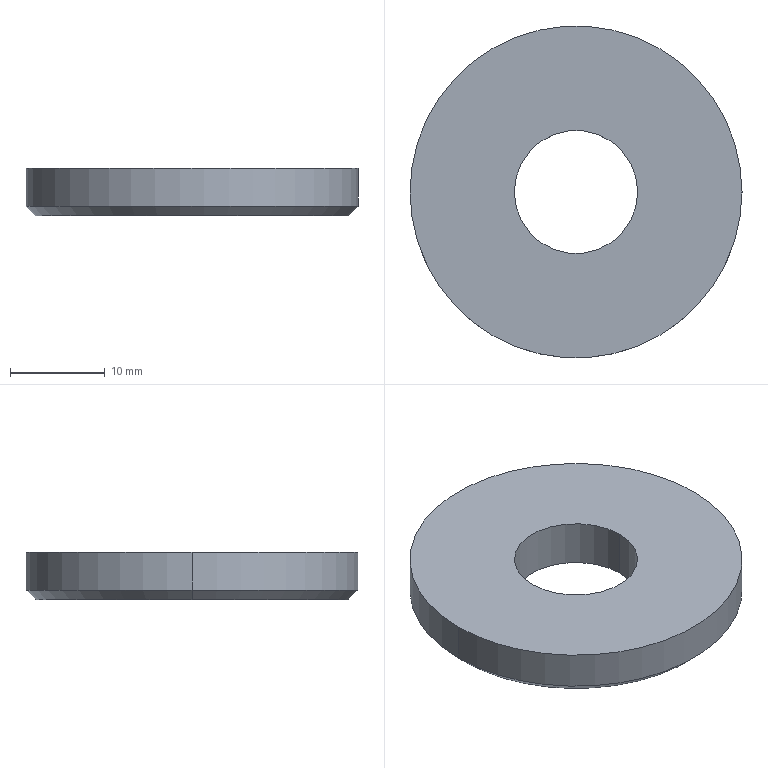Component | SolidWorks | DoubleFilmTransport-1_TensionConnectionAxisPad-1 | 1 solid | 8 faces | box 35 x 35 x 5 mm | volume 4093 mm3 | cylinder 4 | cone 2 | plane 2 | commonest cylinder face diameters 13 x2 35 x2
build123d program:
from build123d import *


with BuildPart() as part:
    # Sketch1 → Revolve1 (revolve)
    with BuildSketch(Plane.XY, mode=Mode.PRIVATE) as revolve1_sk:
        Polygon((5, 16.5), (4, 17.5), (0, 17.5), (0, 6.5), (5, 6.5), align=None)
    revolve(revolve1_sk.sketch.rotate(Axis((0, 0, 0), (1, 0, 0)), 270), axis=Axis((0, 0, 0), (1, 0, 0)))


solid = part.part

# Placed as in the assembly
solid = solid.moved(Location((-384.677, 265.373, 76), (0, 90, 0)))
STEP:
#1=COLOUR_RGB('',0.7922,0.8196,0.9333);
#2=FILL_AREA_STYLE_COLOUR('',#1);
#3=FILL_AREA_STYLE('',(#2));
#4=SURFACE_STYLE_FILL_AREA(#3);
#5=SURFACE_SIDE_STYLE('',(#4));
#6=SURFACE_STYLE_USAGE(.BOTH.,#5);
#7=PRESENTATION_STYLE_ASSIGNMENT((#6));
#8=CARTESIAN_POINT('',(-14.889,10.448,2.992));
#9=VERTEX_POINT('',#8);
#10=CARTESIAN_POINT('',(-15.401,10.448,2.992));
#11=VERTEX_POINT('',#10);
#12=CARTESIAN_POINT('',(-15.145,10.448,2.992));
#13=DIRECTION('',(0.,0.,-1.));
#14=DIRECTION('',(-1.,0.,0.));
#15=AXIS2_PLACEMENT_3D('',#12,#13,#14);
#16=CIRCLE('',#15,0.2559);
#17=EDGE_CURVE('',#9,#11,#16,.T.);
#18=ORIENTED_EDGE('',*,*,#17,.F.);
#19=CARTESIAN_POINT('',(-14.889,10.448,2.795));
#20=VERTEX_POINT('',#19);
#21=CARTESIAN_POINT('',(-14.889,10.448,2.992));
#22=DIRECTION('',(0.,0.,-1.));
#23=VECTOR('',#22,39.37);
#24=LINE('',#21,#23);
#25=EDGE_CURVE('',#9,#20,#24,.T.);
#26=ORIENTED_EDGE('',*,*,#25,.T.);
#27=CARTESIAN_POINT('',(-15.401,10.448,2.795));
#28=VERTEX_POINT('',#27);
#29=CARTESIAN_POINT('',(-15.145,10.448,2.795));
#30=DIRECTION('',(0.,0.,-1.));
#31=DIRECTION('',(-1.,0.,0.));
#32=AXIS2_PLACEMENT_3D('',#29,#30,#31);
#33=CIRCLE('',#32,0.2559);
#34=EDGE_CURVE('',#20,#28,#33,.T.);
#35=ORIENTED_EDGE('',*,*,#34,.T.);
#36=CARTESIAN_POINT('',(-15.401,10.448,2.992));
#37=DIRECTION('',(0.,0.,-1.));
#38=VECTOR('',#37,39.37);
#39=LINE('',#36,#38);
#40=EDGE_CURVE('',#11,#28,#39,.T.);
#41=ORIENTED_EDGE('',*,*,#40,.F.);
#42=EDGE_LOOP('',(#18,#26,#35,#41));
#43=FACE_OUTER_BOUND('',#42,.T.);
#44=CARTESIAN_POINT('',(-15.145,10.448,2.992));
#45=DIRECTION('',(0.,0.,-1.));
#46=DIRECTION('',(-1.,0.,0.));
#47=AXIS2_PLACEMENT_3D('',#44,#45,#46);
#48=CYLINDRICAL_SURFACE('',#47,0.2559);
#49=ADVANCED_FACE('',(#43),#48,.F.);
#50=CARTESIAN_POINT('',(-15.834,10.448,2.992));
#51=VERTEX_POINT('',#50);
#52=CARTESIAN_POINT('',(-14.456,10.448,2.992));
#53=VERTEX_POINT('',#52);
#54=CARTESIAN_POINT('',(-15.145,10.448,2.992));
#55=DIRECTION('',(0.,0.,-1.));
#56=DIRECTION('',(-1.,0.,0.));
#57=AXIS2_PLACEMENT_3D('',#54,#55,#56);
#58=CIRCLE('',#57,0.689);
#59=EDGE_CURVE('',#51,#53,#58,.T.);
#60=ORIENTED_EDGE('',*,*,#59,.T.);
#61=CARTESIAN_POINT('',(-14.456,10.448,2.835));
#62=VERTEX_POINT('',#61);
#63=CARTESIAN_POINT('',(-14.456,10.448,2.992));
#64=DIRECTION('',(0.,0.,-1.));
#65=VECTOR('',#64,39.37);
#66=LINE('',#63,#65);
#67=EDGE_CURVE('',#53,#62,#66,.T.);
#68=ORIENTED_EDGE('',*,*,#67,.T.);
#69=CARTESIAN_POINT('',(-15.834,10.448,2.835));
#70=VERTEX_POINT('',#69);
#71=CARTESIAN_POINT('',(-15.145,10.448,2.835));
#72=DIRECTION('',(0.,0.,-1.));
#73=DIRECTION('',(-1.,0.,0.));
#74=AXIS2_PLACEMENT_3D('',#71,#72,#73);
#75=CIRCLE('',#74,0.689);
#76=EDGE_CURVE('',#70,#62,#75,.T.);
#77=ORIENTED_EDGE('',*,*,#76,.F.);
#78=CARTESIAN_POINT('',(-15.834,10.448,2.992));
#79=DIRECTION('',(0.,0.,-1.));
#80=VECTOR('',#79,39.37);
#81=LINE('',#78,#80);
#82=EDGE_CURVE('',#51,#70,#81,.T.);
#83=ORIENTED_EDGE('',*,*,#82,.F.);
#84=EDGE_LOOP('',(#60,#68,#77,#83));
#85=FACE_OUTER_BOUND('',#84,.T.);
#86=CARTESIAN_POINT('',(-15.145,10.448,2.992));
#87=DIRECTION('',(0.,0.,-1.));
#88=DIRECTION('',(-1.,0.,0.));
#89=AXIS2_PLACEMENT_3D('',#86,#87,#88);
#90=CYLINDRICAL_SURFACE('',#89,0.689);
#91=ADVANCED_FACE('',(#85),#90,.T.);
#92=CARTESIAN_POINT('',(-15.794,10.448,2.795));
#93=VERTEX_POINT('',#92);
#94=CARTESIAN_POINT('',(-14.495,10.448,2.795));
#95=VERTEX_POINT('',#94);
#96=CARTESIAN_POINT('',(-15.145,10.448,2.795));
#97=DIRECTION('',(0.,0.,-1.));
#98=DIRECTION('',(-1.,0.,0.));
#99=AXIS2_PLACEMENT_3D('',#96,#97,#98);
#100=CIRCLE('',#99,0.6496);
#101=EDGE_CURVE('',#93,#95,#100,.T.);
#102=ORIENTED_EDGE('',*,*,#101,.F.);
#103=CARTESIAN_POINT('',(-15.794,10.448,2.795));
#104=DIRECTION('',(-0.7071,0.,0.7071));
#105=VECTOR('',#104,39.37);
#106=LINE('',#103,#105);
#107=EDGE_CURVE('',#93,#70,#106,.T.);
#108=ORIENTED_EDGE('',*,*,#107,.T.);
#109=ORIENTED_EDGE('',*,*,#76,.T.);
#110=CARTESIAN_POINT('',(-14.495,10.448,2.795));
#111=DIRECTION('',(0.7071,0.,0.7071));
#112=VECTOR('',#111,39.37);
#113=LINE('',#110,#112);
#114=EDGE_CURVE('',#95,#62,#113,.T.);
#115=ORIENTED_EDGE('',*,*,#114,.F.);
#116=EDGE_LOOP('',(#102,#108,#109,#115));
#117=FACE_OUTER_BOUND('',#116,.T.);
#118=CARTESIAN_POINT('',(-15.145,10.448,2.795));
#119=DIRECTION('',(0.,0.,1.));
#120=DIRECTION('',(1.,0.,0.));
#121=AXIS2_PLACEMENT_3D('',#118,#119,#120);
#122=CONICAL_SURFACE('',#121,0.6496,0.7854);
#123=ADVANCED_FACE('',(#117),#122,.T.);
#124=CARTESIAN_POINT('',(-15.145,10.448,2.795));
#125=DIRECTION('',(0.,0.,-1.));
#126=DIRECTION('',(-1.,0.,0.));
#127=AXIS2_PLACEMENT_3D('',#124,#125,#126);
#128=CIRCLE('',#127,0.6496);
#129=EDGE_CURVE('',#95,#93,#128,.T.);
#130=ORIENTED_EDGE('',*,*,#129,.T.);
#131=ORIENTED_EDGE('',*,*,#101,.T.);
#132=EDGE_LOOP('',(#130,#131));
#133=FACE_OUTER_BOUND('',#132,.T.);
#134=CARTESIAN_POINT('',(-15.145,10.448,2.795));
#135=DIRECTION('',(0.,0.,-1.));
#136=DIRECTION('',(-1.,0.,0.));
#137=AXIS2_PLACEMENT_3D('',#134,#135,#136);
#138=CIRCLE('',#137,0.2559);
#139=EDGE_CURVE('',#28,#20,#138,.T.);
#140=ORIENTED_EDGE('',*,*,#139,.F.);
#141=ORIENTED_EDGE('',*,*,#34,.F.);
#142=EDGE_LOOP('',(#140,#141));
#143=FACE_BOUND('',#142,.T.);
#144=CARTESIAN_POINT('',(-15.145,10.704,2.795));
#145=DIRECTION('',(0.,0.,-1.));
#146=DIRECTION('',(-1.,0.,0.));
#147=AXIS2_PLACEMENT_3D('',#144,#145,#146);
#148=PLANE('',#147);
#149=ADVANCED_FACE('',(#133,#143),#148,.T.);
#150=ORIENTED_EDGE('',*,*,#107,.F.);
#151=ORIENTED_EDGE('',*,*,#129,.F.);
#152=ORIENTED_EDGE('',*,*,#114,.T.);
#153=CARTESIAN_POINT('',(-15.145,10.448,2.835));
#154=DIRECTION('',(0.,0.,-1.));
#155=DIRECTION('',(-1.,0.,0.));
#156=AXIS2_PLACEMENT_3D('',#153,#154,#155);
#157=CIRCLE('',#156,0.689);
#158=EDGE_CURVE('',#62,#70,#157,.T.);
#159=ORIENTED_EDGE('',*,*,#158,.T.);
#160=EDGE_LOOP('',(#150,#151,#152,#159));
#161=FACE_OUTER_BOUND('',#160,.T.);
#162=CARTESIAN_POINT('',(-15.145,10.448,2.795));
#163=DIRECTION('',(0.,0.,1.));
#164=DIRECTION('',(1.,0.,0.));
#165=AXIS2_PLACEMENT_3D('',#162,#163,#164);
#166=CONICAL_SURFACE('',#165,0.6496,0.7854);
#167=ADVANCED_FACE('',(#161),#166,.T.);
#168=ORIENTED_EDGE('',*,*,#67,.F.);
#169=CARTESIAN_POINT('',(-15.145,10.448,2.992));
#170=DIRECTION('',(0.,0.,-1.));
#171=DIRECTION('',(-1.,0.,0.));
#172=AXIS2_PLACEMENT_3D('',#169,#170,#171);
#173=CIRCLE('',#172,0.689);
#174=EDGE_CURVE('',#53,#51,#173,.T.);
#175=ORIENTED_EDGE('',*,*,#174,.T.);
#176=ORIENTED_EDGE('',*,*,#82,.T.);
#177=ORIENTED_EDGE('',*,*,#158,.F.);
#178=EDGE_LOOP('',(#168,#175,#176,#177));
#179=FACE_OUTER_BOUND('',#178,.T.);
#180=CARTESIAN_POINT('',(-15.145,10.448,2.992));
#181=DIRECTION('',(0.,0.,-1.));
#182=DIRECTION('',(-1.,0.,0.));
#183=AXIS2_PLACEMENT_3D('',#180,#181,#182);
#184=CYLINDRICAL_SURFACE('',#183,0.689);
#185=ADVANCED_FACE('',(#179),#184,.T.);
#186=CARTESIAN_POINT('',(-15.145,10.448,2.992));
#187=DIRECTION('',(0.,0.,-1.));
#188=DIRECTION('',(-1.,0.,0.));
#189=AXIS2_PLACEMENT_3D('',#186,#187,#188);
#190=CIRCLE('',#189,0.2559);
#191=EDGE_CURVE('',#11,#9,#190,.T.);
#192=ORIENTED_EDGE('',*,*,#191,.T.);
#193=ORIENTED_EDGE('',*,*,#17,.T.);
#194=EDGE_LOOP('',(#192,#193));
#195=FACE_BOUND('',#194,.T.);
#196=ORIENTED_EDGE('',*,*,#59,.F.);
#197=ORIENTED_EDGE('',*,*,#174,.F.);
#198=EDGE_LOOP('',(#196,#197));
#199=FACE_OUTER_BOUND('',#198,.T.);
#200=CARTESIAN_POINT('',(-15.145,11.137,2.992));
#201=DIRECTION('',(0.,0.,1.));
#202=DIRECTION('',(1.,0.,0.));
#203=AXIS2_PLACEMENT_3D('',#200,#201,#202);
#204=PLANE('',#203);
#205=ADVANCED_FACE('',(#195,#199),#204,.T.);
#206=ORIENTED_EDGE('',*,*,#25,.F.);
#207=ORIENTED_EDGE('',*,*,#191,.F.);
#208=ORIENTED_EDGE('',*,*,#40,.T.);
#209=ORIENTED_EDGE('',*,*,#139,.T.);
#210=EDGE_LOOP('',(#206,#207,#208,#209));
#211=FACE_OUTER_BOUND('',#210,.T.);
#212=CARTESIAN_POINT('',(-15.145,10.448,2.992));
#213=DIRECTION('',(0.,0.,-1.));
#214=DIRECTION('',(-1.,0.,0.));
#215=AXIS2_PLACEMENT_3D('',#212,#213,#214);
#216=CYLINDRICAL_SURFACE('',#215,0.2559);
#217=ADVANCED_FACE('',(#211),#216,.F.);
#218=CLOSED_SHELL('',(#49,#91,#123,#149,#167,#185,#205,#217));
#219=MANIFOLD_SOLID_BREP('',#218);
#220=STYLED_ITEM('',(#7),#219);
#221=PRESENTATION_LAYER_ASSIGNMENT('','',(#220));
#222=(LENGTH_UNIT()NAMED_UNIT(*)SI_UNIT($,.METRE.));
#223=LENGTH_MEASURE_WITH_UNIT(LENGTH_MEASURE(0.0254),#222);
#224=DIMENSIONAL_EXPONENTS(1.,0.,0.,0.,0.,0.,0.);
#225=(CONVERSION_BASED_UNIT('',#223)LENGTH_UNIT()NAMED_UNIT(#224));
#226=UNCERTAINTY_MEASURE_WITH_UNIT(LENGTH_MEASURE(0.00001),#225,'','');
#227=(NAMED_UNIT(*)PLANE_ANGLE_UNIT()SI_UNIT($,.RADIAN.));
#228=(NAMED_UNIT(*)SI_UNIT($,.STERADIAN.)SOLID_ANGLE_UNIT());
#229=(GEOMETRIC_REPRESENTATION_CONTEXT(3)GLOBAL_UNCERTAINTY_ASSIGNED_CONTEXT((#226))GLOBAL_UNIT_ASSIGNED_CONTEXT((#225,#227,#228))REPRESENTATION_CONTEXT('',''));
#230=MECHANICAL_DESIGN_GEOMETRIC_PRESENTATION_REPRESENTATION('',(#220),#229);
#231=CARTESIAN_POINT('',(0.,0.,0.));
#232=DIRECTION('',(0.,0.,1.));
#233=DIRECTION('',(1.,0.,0.));
#234=AXIS2_PLACEMENT_3D('',#231,#232,#233);
#235=(LENGTH_UNIT()NAMED_UNIT(*)SI_UNIT($,.METRE.));
#236=LENGTH_MEASURE_WITH_UNIT(LENGTH_MEASURE(0.0254),#235);
#237=DIMENSIONAL_EXPONENTS(1.,0.,0.,0.,0.,0.,0.);
#238=(CONVERSION_BASED_UNIT('',#236)LENGTH_UNIT()NAMED_UNIT(#237));
#239=UNCERTAINTY_MEASURE_WITH_UNIT(LENGTH_MEASURE(0.00001),#238,'','');
#240=(NAMED_UNIT(*)PLANE_ANGLE_UNIT()SI_UNIT($,.RADIAN.));
#241=(NAMED_UNIT(*)SI_UNIT($,.STERADIAN.)SOLID_ANGLE_UNIT());
#242=(GEOMETRIC_REPRESENTATION_CONTEXT(3)GLOBAL_UNCERTAINTY_ASSIGNED_CONTEXT((#239))GLOBAL_UNIT_ASSIGNED_CONTEXT((#238,#240,#241))REPRESENTATION_CONTEXT('',''));
#243=ADVANCED_BREP_SHAPE_REPRESENTATION('',(#219,#234),#242);